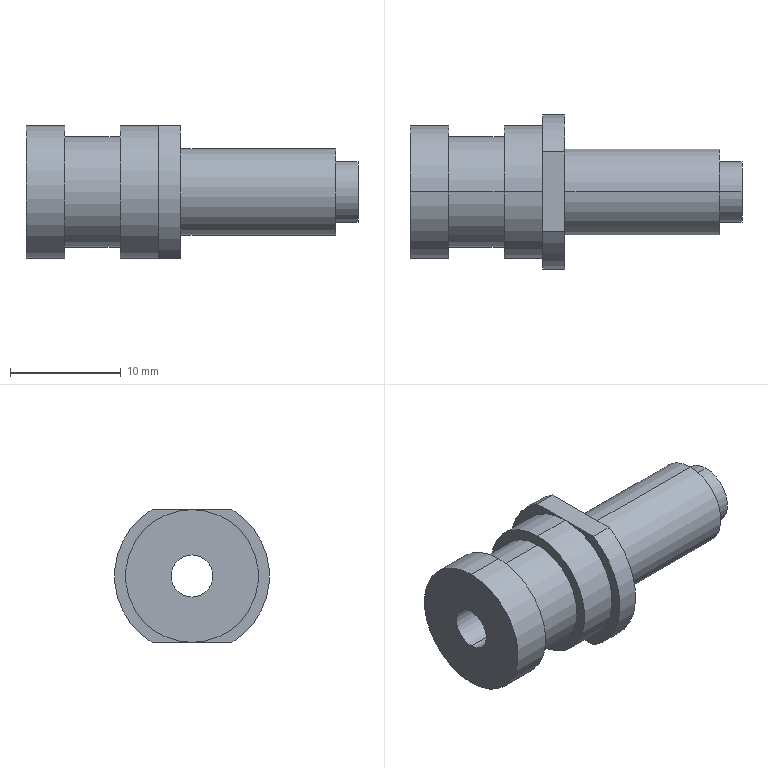Component | SolidWorks | Connector-1 | 1 solid | 24 faces | box 30 x 14 x 12 mm | volume 1849 mm3 | cylinder 14 | plane 10 | commonest cylinder face diameters 12 x4 10 x2 5.5 x2 3.8 x2 7.8 x2 14 x2
build123d program:
from build123d import *

# Parameters (mm, degrees)
SKETCH1_R           = 3.9
BOSS_EXTRUDE1_DEPTH = 16
SKETCH2_R           = 7
BOSS_EXTRUDE2_DEPTH = 14
SKETCH3_R           = 1.9
CUT_EXTRUDE1_DEPTH  = 32.591
CHAMFER1_SIZE       = 1
CUT_EXTRUDE2_START  = -12
SKETCH4_R           = 7
SKETCH4_R_2         = 6
CUT_EXTRUDE2_DEPTH  = 12
SKETCH6_R           = 4.5
SKETCH6_R_2         = 2.75
CUT_EXTRUDE4_DEPTH  = 2
SKETCH8_W           = 1
SKETCH8_H           = 5
CUT_EXTRUDE5_DEPTH  = 19.815


with BuildPart() as part:
    # Sketch1 → Boss-Extrude1 (new body)
    with BuildSketch(Plane.XY):
        Circle(SKETCH1_R)
    extrude(amount=BOSS_EXTRUDE1_DEPTH)

    # Sketch2 → Boss-Extrude2 (add)
    with BuildSketch(Plane.XY.offset(16)):
        Circle(SKETCH2_R)
    extrude(amount=BOSS_EXTRUDE2_DEPTH)

    # Sketch3 → Cut-Extrude1 (cut, through all)
    with BuildSketch(Plane(origin=(0, 0, 0), x_dir=(-1, 0, 0), z_dir=(0, 0, -1))):
        Circle(SKETCH3_R)
    extrude(amount=-CUT_EXTRUDE1_DEPTH, mode=Mode.SUBTRACT)

    # Chamfer1
    chamfer1_edges = [part.edges().sort_by_distance(p)[0] for p in [
        (-3.9, 0, 0),
    ]]
    chamfer(chamfer1_edges, length=CHAMFER1_SIZE)

    # Sketch4 → Cut-Extrude2 (cut)
    with BuildSketch(Plane.XY.offset(30).offset(CUT_EXTRUDE2_START)):
        Circle(SKETCH4_R)
        Circle(SKETCH4_R_2, mode=Mode.SUBTRACT)
    extrude(amount=CUT_EXTRUDE2_DEPTH, mode=Mode.SUBTRACT)

    # Sketch6 → Cut-Extrude4 (cut)
    with BuildSketch(Plane(origin=(0, 0, 0), x_dir=(-1, 0, 0), z_dir=(0, 0, -1))):
        Circle(SKETCH6_R)
        Circle(SKETCH6_R_2, mode=Mode.SUBTRACT)
    extrude(amount=-CUT_EXTRUDE4_DEPTH, mode=Mode.SUBTRACT)

    # Sketch8 → Cut-Revolve1 (revolve, cut)
    with BuildSketch(Plane(origin=(0, 0, 0), x_dir=(1, 0, 0), z_dir=(0, 1, 0)), mode=Mode.PRIVATE) as cut_revolve1_sk:
        with Locations((-5.5, -24)):
            Rectangle(SKETCH8_W, SKETCH8_H)
    revolve(cut_revolve1_sk.sketch.rotate(Axis((0, 0, 30), (0, 0, -1)), 180), axis=Axis((0, 0, 30), (0, 0, -1)), mode=Mode.SUBTRACT)

    # Sketch9 → Cut-Extrude5 (cut, through all)
    with BuildSketch(Plane(origin=(0, 0, 16), x_dir=(-1, 0, 0), z_dir=(0, 0, -1))):
        with BuildLine():
            Line((-6, 3.606), (-6, -3.606))
            ThreePointArc((-6, -3.606), (-7, 0), (-6, 3.606))
        make_face()
        with BuildLine():
            Line((6, 3.606), (6, -3.606))
            ThreePointArc((6, -3.606), (7, 0), (6, 3.606))
        make_face()
    extrude(amount=-CUT_EXTRUDE5_DEPTH, mode=Mode.SUBTRACT)


solid = part.part

# Placed as in the assembly
solid = solid.moved(Location((20.76, 74.679, 11), (0, -90, 0)))
STEP:
#1=CARTESIAN_POINT('',(-0.02914,2.94,0.6299));
#2=VERTEX_POINT('',#1);
#3=CARTESIAN_POINT('',(-0.02914,2.94,0.2362));
#4=VERTEX_POINT('',#3);
#5=CARTESIAN_POINT('',(-0.02914,2.94,0.4331));
#6=DIRECTION('',(-1.,-0.,-0.));
#7=DIRECTION('',(-0.,0.,1.));
#8=AXIS2_PLACEMENT_3D('',#5,#6,#7);
#9=CIRCLE('',#8,0.1969);
#10=EDGE_CURVE('',#2,#4,#9,.T.);
#11=ORIENTED_EDGE('',*,*,#10,.T.);
#12=CARTESIAN_POINT('',(-0.226,2.94,0.2362));
#13=VERTEX_POINT('',#12);
#14=CARTESIAN_POINT('',(-0.3638,2.94,0.2362));
#15=DIRECTION('',(-1.,-0.,-0.));
#16=VECTOR('',#15,39.37);
#17=LINE('',#14,#16);
#18=EDGE_CURVE('',#4,#13,#17,.T.);
#19=ORIENTED_EDGE('',*,*,#18,.T.);
#20=CARTESIAN_POINT('',(-0.226,2.94,0.6299));
#21=VERTEX_POINT('',#20);
#22=CARTESIAN_POINT('',(-0.226,2.94,0.4331));
#23=DIRECTION('',(-1.,-0.,-0.));
#24=DIRECTION('',(-0.,0.,1.));
#25=AXIS2_PLACEMENT_3D('',#22,#23,#24);
#26=CIRCLE('',#25,0.1969);
#27=EDGE_CURVE('',#21,#13,#26,.T.);
#28=ORIENTED_EDGE('',*,*,#27,.F.);
#29=CARTESIAN_POINT('',(-0.3638,2.94,0.6299));
#30=DIRECTION('',(-1.,-0.,-0.));
#31=VECTOR('',#30,39.37);
#32=LINE('',#29,#31);
#33=EDGE_CURVE('',#2,#21,#32,.T.);
#34=ORIENTED_EDGE('',*,*,#33,.F.);
#35=EDGE_LOOP('',(#11,#19,#28,#34));
#36=FACE_OUTER_BOUND('',#35,.T.);
#37=CARTESIAN_POINT('',(-0.3638,2.94,0.4331));
#38=DIRECTION('',(-1.,-0.,-0.));
#39=DIRECTION('',(-0.,0.,1.));
#40=AXIS2_PLACEMENT_3D('',#37,#38,#39);
#41=CYLINDRICAL_SURFACE('',#40,0.1969);
#42=ADVANCED_FACE('',(#36),#41,.T.);
#43=CARTESIAN_POINT('',(0.7386,2.94,0.3248));
#44=VERTEX_POINT('',#43);
#45=CARTESIAN_POINT('',(0.7386,2.94,0.5413));
#46=VERTEX_POINT('',#45);
#47=CARTESIAN_POINT('',(0.7386,2.94,0.4331));
#48=DIRECTION('',(1.,0.,0.));
#49=DIRECTION('',(0.,0.,-1.));
#50=AXIS2_PLACEMENT_3D('',#47,#48,#49);
#51=CIRCLE('',#50,0.1083);
#52=EDGE_CURVE('',#44,#46,#51,.T.);
#53=ORIENTED_EDGE('',*,*,#52,.T.);
#54=CARTESIAN_POINT('',(0.8173,2.94,0.5413));
#55=VERTEX_POINT('',#54);
#56=CARTESIAN_POINT('',(0.7386,2.94,0.5413));
#57=DIRECTION('',(1.,0.,0.));
#58=VECTOR('',#57,39.37);
#59=LINE('',#56,#58);
#60=EDGE_CURVE('',#46,#55,#59,.T.);
#61=ORIENTED_EDGE('',*,*,#60,.T.);
#62=CARTESIAN_POINT('',(0.8173,2.94,0.3248));
#63=VERTEX_POINT('',#62);
#64=CARTESIAN_POINT('',(0.8173,2.94,0.4331));
#65=DIRECTION('',(1.,0.,0.));
#66=DIRECTION('',(0.,0.,-1.));
#67=AXIS2_PLACEMENT_3D('',#64,#65,#66);
#68=CIRCLE('',#67,0.1083);
#69=EDGE_CURVE('',#63,#55,#68,.T.);
#70=ORIENTED_EDGE('',*,*,#69,.F.);
#71=CARTESIAN_POINT('',(0.7386,2.94,0.3248));
#72=DIRECTION('',(1.,0.,0.));
#73=VECTOR('',#72,39.37);
#74=LINE('',#71,#73);
#75=EDGE_CURVE('',#44,#63,#74,.T.);
#76=ORIENTED_EDGE('',*,*,#75,.F.);
#77=EDGE_LOOP('',(#53,#61,#70,#76));
#78=FACE_OUTER_BOUND('',#77,.T.);
#79=CARTESIAN_POINT('',(0.7386,2.94,0.4331));
#80=DIRECTION('',(1.,0.,0.));
#81=DIRECTION('',(0.,0.,-1.));
#82=AXIS2_PLACEMENT_3D('',#79,#80,#81);
#83=CYLINDRICAL_SURFACE('',#82,0.1083);
#84=ADVANCED_FACE('',(#78),#83,.T.);
#85=CARTESIAN_POINT('',(-0.3638,2.94,0.5079));
#86=VERTEX_POINT('',#85);
#87=CARTESIAN_POINT('',(-0.3638,2.94,0.3583));
#88=VERTEX_POINT('',#87);
#89=CARTESIAN_POINT('',(-0.3638,2.94,0.4331));
#90=DIRECTION('',(1.,0.,0.));
#91=DIRECTION('',(0.,0.,-1.));
#92=AXIS2_PLACEMENT_3D('',#89,#90,#91);
#93=CIRCLE('',#92,0.0748);
#94=EDGE_CURVE('',#86,#88,#93,.T.);
#95=ORIENTED_EDGE('',*,*,#94,.F.);
#96=CARTESIAN_POINT('',(0.8173,2.94,0.5079));
#97=VERTEX_POINT('',#96);
#98=CARTESIAN_POINT('',(-0.3638,2.94,0.5079));
#99=DIRECTION('',(1.,0.,0.));
#100=VECTOR('',#99,39.37);
#101=LINE('',#98,#100);
#102=EDGE_CURVE('',#86,#97,#101,.T.);
#103=ORIENTED_EDGE('',*,*,#102,.T.);
#104=CARTESIAN_POINT('',(0.8173,2.94,0.3583));
#105=VERTEX_POINT('',#104);
#106=CARTESIAN_POINT('',(0.8173,2.94,0.4331));
#107=DIRECTION('',(1.,0.,0.));
#108=DIRECTION('',(0.,0.,-1.));
#109=AXIS2_PLACEMENT_3D('',#106,#107,#108);
#110=CIRCLE('',#109,0.0748);
#111=EDGE_CURVE('',#97,#105,#110,.T.);
#112=ORIENTED_EDGE('',*,*,#111,.T.);
#113=CARTESIAN_POINT('',(-0.3638,2.94,0.3583));
#114=DIRECTION('',(1.,0.,0.));
#115=VECTOR('',#114,39.37);
#116=LINE('',#113,#115);
#117=EDGE_CURVE('',#88,#105,#116,.T.);
#118=ORIENTED_EDGE('',*,*,#117,.F.);
#119=EDGE_LOOP('',(#95,#103,#112,#118));
#120=FACE_OUTER_BOUND('',#119,.T.);
#121=CARTESIAN_POINT('',(-0.3638,2.94,0.4331));
#122=DIRECTION('',(1.,0.,0.));
#123=DIRECTION('',(0.,0.,-1.));
#124=AXIS2_PLACEMENT_3D('',#121,#122,#123);
#125=CYLINDRICAL_SURFACE('',#124,0.0748);
#126=ADVANCED_FACE('',(#120),#125,.F.);
#127=CARTESIAN_POINT('',(0.1874,2.94,0.5866));
#128=VERTEX_POINT('',#127);
#129=CARTESIAN_POINT('',(0.1874,2.94,0.2795));
#130=VERTEX_POINT('',#129);
#131=CARTESIAN_POINT('',(0.1874,2.94,0.4331));
#132=DIRECTION('',(-1.,-0.,-0.));
#133=DIRECTION('',(-0.,0.,1.));
#134=AXIS2_PLACEMENT_3D('',#131,#132,#133);
#135=CIRCLE('',#134,0.1535);
#136=EDGE_CURVE('',#128,#130,#135,.T.);
#137=ORIENTED_EDGE('',*,*,#136,.F.);
#138=CARTESIAN_POINT('',(0.7386,2.94,0.5866));
#139=VERTEX_POINT('',#138);
#140=CARTESIAN_POINT('',(0.1874,2.94,0.5866));
#141=DIRECTION('',(1.,0.,0.));
#142=VECTOR('',#141,39.37);
#143=LINE('',#140,#142);
#144=EDGE_CURVE('',#128,#139,#143,.T.);
#145=ORIENTED_EDGE('',*,*,#144,.T.);
#146=CARTESIAN_POINT('',(0.7386,2.94,0.2795));
#147=VERTEX_POINT('',#146);
#148=CARTESIAN_POINT('',(0.7386,2.94,0.4331));
#149=DIRECTION('',(1.,0.,0.));
#150=DIRECTION('',(0.,0.,-1.));
#151=AXIS2_PLACEMENT_3D('',#148,#149,#150);
#152=CIRCLE('',#151,0.1535);
#153=EDGE_CURVE('',#147,#139,#152,.T.);
#154=ORIENTED_EDGE('',*,*,#153,.F.);
#155=CARTESIAN_POINT('',(0.1874,2.94,0.2795));
#156=DIRECTION('',(1.,0.,0.));
#157=VECTOR('',#156,39.37);
#158=LINE('',#155,#157);
#159=EDGE_CURVE('',#130,#147,#158,.T.);
#160=ORIENTED_EDGE('',*,*,#159,.F.);
#161=EDGE_LOOP('',(#137,#145,#154,#160));
#162=FACE_OUTER_BOUND('',#161,.T.);
#163=CARTESIAN_POINT('',(0.1874,2.94,0.4331));
#164=DIRECTION('',(1.,0.,0.));
#165=DIRECTION('',(0.,0.,-1.));
#166=AXIS2_PLACEMENT_3D('',#163,#164,#165);
#167=CYLINDRICAL_SURFACE('',#166,0.1535);
#168=ADVANCED_FACE('',(#162),#167,.T.);
#169=CARTESIAN_POINT('',(0.1087,2.94,0.6693));
#170=VERTEX_POINT('',#169);
#171=CARTESIAN_POINT('',(0.1087,2.94,0.1969));
#172=VERTEX_POINT('',#171);
#173=CARTESIAN_POINT('',(0.1087,2.94,0.4331));
#174=DIRECTION('',(-1.,-0.,-0.));
#175=DIRECTION('',(-0.,0.,1.));
#176=AXIS2_PLACEMENT_3D('',#173,#174,#175);
#177=CIRCLE('',#176,0.2362);
#178=EDGE_CURVE('',#170,#172,#177,.T.);
#179=ORIENTED_EDGE('',*,*,#178,.T.);
#180=CARTESIAN_POINT('',(-0.02914,2.94,0.1969));
#181=VERTEX_POINT('',#180);
#182=CARTESIAN_POINT('',(0.1087,2.94,0.1969));
#183=DIRECTION('',(-1.,-0.,-0.));
#184=VECTOR('',#183,39.37);
#185=LINE('',#182,#184);
#186=EDGE_CURVE('',#172,#181,#185,.T.);
#187=ORIENTED_EDGE('',*,*,#186,.T.);
#188=CARTESIAN_POINT('',(-0.02914,2.94,0.6693));
#189=VERTEX_POINT('',#188);
#190=CARTESIAN_POINT('',(-0.02914,2.94,0.4331));
#191=DIRECTION('',(-1.,-0.,-0.));
#192=DIRECTION('',(-0.,0.,1.));
#193=AXIS2_PLACEMENT_3D('',#190,#191,#192);
#194=CIRCLE('',#193,0.2362);
#195=EDGE_CURVE('',#189,#181,#194,.T.);
#196=ORIENTED_EDGE('',*,*,#195,.F.);
#197=CARTESIAN_POINT('',(0.1087,2.94,0.6693));
#198=DIRECTION('',(-1.,-0.,-0.));
#199=VECTOR('',#198,39.37);
#200=LINE('',#197,#199);
#201=EDGE_CURVE('',#170,#189,#200,.T.);
#202=ORIENTED_EDGE('',*,*,#201,.F.);
#203=EDGE_LOOP('',(#179,#187,#196,#202));
#204=FACE_OUTER_BOUND('',#203,.T.);
#205=CARTESIAN_POINT('',(0.1087,2.94,0.4331));
#206=DIRECTION('',(-1.,-0.,-0.));
#207=DIRECTION('',(-0.,0.,1.));
#208=AXIS2_PLACEMENT_3D('',#205,#206,#207);
#209=CYLINDRICAL_SURFACE('',#208,0.2362);
#210=ADVANCED_FACE('',(#204),#209,.T.);
#211=CARTESIAN_POINT('',(-0.226,2.94,0.6693));
#212=VERTEX_POINT('',#211);
#213=CARTESIAN_POINT('',(-0.226,2.94,0.1969));
#214=VERTEX_POINT('',#213);
#215=CARTESIAN_POINT('',(-0.226,2.94,0.4331));
#216=DIRECTION('',(-1.,-0.,-0.));
#217=DIRECTION('',(-0.,0.,1.));
#218=AXIS2_PLACEMENT_3D('',#215,#216,#217);
#219=CIRCLE('',#218,0.2362);
#220=EDGE_CURVE('',#212,#214,#219,.T.);
#221=ORIENTED_EDGE('',*,*,#220,.T.);
#222=CARTESIAN_POINT('',(-0.3638,2.94,0.1969));
#223=VERTEX_POINT('',#222);
#224=CARTESIAN_POINT('',(0.1087,2.94,0.1969));
#225=DIRECTION('',(-1.,-0.,-0.));
#226=VECTOR('',#225,39.37);
#227=LINE('',#224,#226);
#228=EDGE_CURVE('',#214,#223,#227,.T.);
#229=ORIENTED_EDGE('',*,*,#228,.T.);
#230=CARTESIAN_POINT('',(-0.3638,2.94,0.6693));
#231=VERTEX_POINT('',#230);
#232=CARTESIAN_POINT('',(-0.3638,2.94,0.4331));
#233=DIRECTION('',(-1.,-0.,-0.));
#234=DIRECTION('',(-0.,0.,1.));
#235=AXIS2_PLACEMENT_3D('',#232,#233,#234);
#236=CIRCLE('',#235,0.2362);
#237=EDGE_CURVE('',#231,#223,#236,.T.);
#238=ORIENTED_EDGE('',*,*,#237,.F.);
#239=CARTESIAN_POINT('',(0.1087,2.94,0.6693));
#240=DIRECTION('',(-1.,-0.,-0.));
#241=VECTOR('',#240,39.37);
#242=LINE('',#239,#241);
#243=EDGE_CURVE('',#212,#231,#242,.T.);
#244=ORIENTED_EDGE('',*,*,#243,.F.);
#245=EDGE_LOOP('',(#221,#229,#238,#244));
#246=FACE_OUTER_BOUND('',#245,.T.);
#247=CARTESIAN_POINT('',(0.1087,2.94,0.4331));
#248=DIRECTION('',(-1.,-0.,-0.));
#249=DIRECTION('',(-0.,0.,1.));
#250=AXIS2_PLACEMENT_3D('',#247,#248,#249);
#251=CYLINDRICAL_SURFACE('',#250,0.2362);
#252=ADVANCED_FACE('',(#246),#251,.T.);
#253=CARTESIAN_POINT('',(0.1087,2.798,0.1969));
#254=VERTEX_POINT('',#253);
#255=CARTESIAN_POINT('',(0.1087,2.798,0.6693));
#256=VERTEX_POINT('',#255);
#257=CARTESIAN_POINT('',(0.1087,2.94,0.4331));
#258=DIRECTION('',(-1.,-0.,-0.));
#259=DIRECTION('',(-0.,0.,1.));
#260=AXIS2_PLACEMENT_3D('',#257,#258,#259);
#261=CIRCLE('',#260,0.2756);
#262=EDGE_CURVE('',#254,#256,#261,.T.);
#263=ORIENTED_EDGE('',*,*,#262,.F.);
#264=CARTESIAN_POINT('',(0.1874,2.798,0.1969));
#265=VERTEX_POINT('',#264);
#266=CARTESIAN_POINT('',(-0.3638,2.798,0.1969));
#267=DIRECTION('',(1.,0.,0.));
#268=VECTOR('',#267,39.37);
#269=LINE('',#266,#268);
#270=EDGE_CURVE('',#254,#265,#269,.T.);
#271=ORIENTED_EDGE('',*,*,#270,.T.);
#272=CARTESIAN_POINT('',(0.1874,2.798,0.6693));
#273=VERTEX_POINT('',#272);
#274=CARTESIAN_POINT('',(0.1874,2.94,0.4331));
#275=DIRECTION('',(-1.,-0.,-0.));
#276=DIRECTION('',(-0.,0.,1.));
#277=AXIS2_PLACEMENT_3D('',#274,#275,#276);
#278=CIRCLE('',#277,0.2756);
#279=EDGE_CURVE('',#265,#273,#278,.T.);
#280=ORIENTED_EDGE('',*,*,#279,.T.);
#281=CARTESIAN_POINT('',(-0.3638,2.798,0.6693));
#282=DIRECTION('',(1.,0.,0.));
#283=VECTOR('',#282,39.37);
#284=LINE('',#281,#283);
#285=EDGE_CURVE('',#256,#273,#284,.T.);
#286=ORIENTED_EDGE('',*,*,#285,.F.);
#287=EDGE_LOOP('',(#263,#271,#280,#286));
#288=FACE_OUTER_BOUND('',#287,.T.);
#289=CARTESIAN_POINT('',(-0.3638,2.94,0.4331));
#290=DIRECTION('',(1.,0.,0.));
#291=DIRECTION('',(0.,0.,-1.));
#292=AXIS2_PLACEMENT_3D('',#289,#290,#291);
#293=CYLINDRICAL_SURFACE('',#292,0.2756);
#294=ADVANCED_FACE('',(#288),#293,.T.);
#295=CARTESIAN_POINT('',(0.1087,2.94,0.1969));
#296=DIRECTION('',(-0.,1.,0.));
#297=VECTOR('',#296,39.37);
#298=LINE('',#295,#297);
#299=EDGE_CURVE('',#254,#172,#298,.T.);
#300=ORIENTED_EDGE('',*,*,#299,.F.);
#301=ORIENTED_EDGE('',*,*,#262,.T.);
#302=CARTESIAN_POINT('',(0.1087,2.94,0.6693));
#303=DIRECTION('',(0.,-1.,0.));
#304=VECTOR('',#303,39.37);
#305=LINE('',#302,#304);
#306=EDGE_CURVE('',#170,#256,#305,.T.);
#307=ORIENTED_EDGE('',*,*,#306,.F.);
#308=CARTESIAN_POINT('',(0.1087,2.94,0.4331));
#309=DIRECTION('',(-1.,-0.,-0.));
#310=DIRECTION('',(-0.,0.,1.));
#311=AXIS2_PLACEMENT_3D('',#308,#309,#310);
#312=CIRCLE('',#311,0.2362);
#313=EDGE_CURVE('',#172,#170,#312,.T.);
#314=ORIENTED_EDGE('',*,*,#313,.F.);
#315=EDGE_LOOP('',(#300,#301,#307,#314));
#316=FACE_OUTER_BOUND('',#315,.T.);
#317=CARTESIAN_POINT('',(0.1087,2.94,0.4331));
#318=DIRECTION('',(-1.,-0.,-0.));
#319=DIRECTION('',(-0.,0.,1.));
#320=AXIS2_PLACEMENT_3D('',#317,#318,#319);
#321=PLANE('',#320);
#322=ADVANCED_FACE('',(#316),#321,.T.);
#323=ORIENTED_EDGE('',*,*,#228,.F.);
#324=CARTESIAN_POINT('',(-0.226,2.94,0.4331));
#325=DIRECTION('',(-1.,-0.,-0.));
#326=DIRECTION('',(-0.,0.,1.));
#327=AXIS2_PLACEMENT_3D('',#324,#325,#326);
#328=CIRCLE('',#327,0.2362);
#329=EDGE_CURVE('',#214,#212,#328,.T.);
#330=ORIENTED_EDGE('',*,*,#329,.T.);
#331=ORIENTED_EDGE('',*,*,#243,.T.);
#332=CARTESIAN_POINT('',(-0.3638,2.94,0.4331));
#333=DIRECTION('',(-1.,-0.,-0.));
#334=DIRECTION('',(-0.,0.,1.));
#335=AXIS2_PLACEMENT_3D('',#332,#333,#334);
#336=CIRCLE('',#335,0.2362);
#337=EDGE_CURVE('',#223,#231,#336,.T.);
#338=ORIENTED_EDGE('',*,*,#337,.F.);
#339=EDGE_LOOP('',(#323,#330,#331,#338));
#340=FACE_OUTER_BOUND('',#339,.T.);
#341=CARTESIAN_POINT('',(0.1087,2.94,0.4331));
#342=DIRECTION('',(-1.,-0.,-0.));
#343=DIRECTION('',(-0.,0.,1.));
#344=AXIS2_PLACEMENT_3D('',#341,#342,#343);
#345=CYLINDRICAL_SURFACE('',#344,0.2362);
#346=ADVANCED_FACE('',(#340),#345,.T.);
#347=ORIENTED_EDGE('',*,*,#186,.F.);
#348=ORIENTED_EDGE('',*,*,#313,.T.);
#349=ORIENTED_EDGE('',*,*,#201,.T.);
#350=CARTESIAN_POINT('',(-0.02914,2.94,0.4331));
#351=DIRECTION('',(-1.,-0.,-0.));
#352=DIRECTION('',(-0.,0.,1.));
#353=AXIS2_PLACEMENT_3D('',#350,#351,#352);
#354=CIRCLE('',#353,0.2362);
#355=EDGE_CURVE('',#181,#189,#354,.T.);
#356=ORIENTED_EDGE('',*,*,#355,.F.);
#357=EDGE_LOOP('',(#347,#348,#349,#356));
#358=FACE_OUTER_BOUND('',#357,.T.);
#359=CARTESIAN_POINT('',(0.1087,2.94,0.4331));
#360=DIRECTION('',(-1.,-0.,-0.));
#361=DIRECTION('',(-0.,0.,1.));
#362=AXIS2_PLACEMENT_3D('',#359,#360,#361);
#363=CYLINDRICAL_SURFACE('',#362,0.2362);
#364=ADVANCED_FACE('',(#358),#363,.T.);
#365=ORIENTED_EDGE('',*,*,#144,.F.);
#366=CARTESIAN_POINT('',(0.1874,2.94,0.4331));
#367=DIRECTION('',(-1.,-0.,-0.));
#368=DIRECTION('',(-0.,0.,1.));
#369=AXIS2_PLACEMENT_3D('',#366,#367,#368);
#370=CIRCLE('',#369,0.1535);
#371=EDGE_CURVE('',#130,#128,#370,.T.);
#372=ORIENTED_EDGE('',*,*,#371,.F.);
#373=ORIENTED_EDGE('',*,*,#159,.T.);
#374=CARTESIAN_POINT('',(0.7386,2.94,0.4331));
#375=DIRECTION('',(1.,0.,0.));
#376=DIRECTION('',(0.,0.,-1.));
#377=AXIS2_PLACEMENT_3D('',#374,#375,#376);
#378=CIRCLE('',#377,0.1535);
#379=EDGE_CURVE('',#139,#147,#378,.T.);
#380=ORIENTED_EDGE('',*,*,#379,.F.);
#381=EDGE_LOOP('',(#365,#372,#373,#380));
#382=FACE_OUTER_BOUND('',#381,.T.);
#383=CARTESIAN_POINT('',(0.1874,2.94,0.4331));
#384=DIRECTION('',(1.,0.,0.));
#385=DIRECTION('',(0.,0.,-1.));
#386=AXIS2_PLACEMENT_3D('',#383,#384,#385);
#387=CYLINDRICAL_SURFACE('',#386,0.1535);
#388=ADVANCED_FACE('',(#382),#387,.T.);
#389=CARTESIAN_POINT('',(0.8173,2.94,0.4331));
#390=DIRECTION('',(1.,0.,0.));
#391=DIRECTION('',(0.,0.,-1.));
#392=AXIS2_PLACEMENT_3D('',#389,#390,#391);
#393=CIRCLE('',#392,0.0748);
#394=EDGE_CURVE('',#105,#97,#393,.T.);
#395=ORIENTED_EDGE('',*,*,#394,.F.);
#396=ORIENTED_EDGE('',*,*,#111,.F.);
#397=EDGE_LOOP('',(#395,#396));
#398=FACE_BOUND('',#397,.T.);
#399=ORIENTED_EDGE('',*,*,#69,.T.);
#400=CARTESIAN_POINT('',(0.8173,2.94,0.4331));
#401=DIRECTION('',(1.,0.,0.));
#402=DIRECTION('',(0.,0.,-1.));
#403=AXIS2_PLACEMENT_3D('',#400,#401,#402);
#404=CIRCLE('',#403,0.1083);
#405=EDGE_CURVE('',#55,#63,#404,.T.);
#406=ORIENTED_EDGE('',*,*,#405,.T.);
#407=EDGE_LOOP('',(#399,#406));
#408=FACE_OUTER_BOUND('',#407,.T.);
#409=CARTESIAN_POINT('',(0.8173,2.94,0.4331));
#410=DIRECTION('',(-1.,-0.,-0.));
#411=DIRECTION('',(-0.,0.,1.));
#412=AXIS2_PLACEMENT_3D('',#409,#410,#411);
#413=PLANE('',#412);
#414=ADVANCED_FACE('',(#398,#408),#413,.F.);
#415=CARTESIAN_POINT('',(0.1874,3.082,0.6693));
#416=VERTEX_POINT('',#415);
#417=CARTESIAN_POINT('',(0.1874,3.082,0.1969));
#418=VERTEX_POINT('',#417);
#419=CARTESIAN_POINT('',(0.1874,2.94,0.4331));
#420=DIRECTION('',(-1.,-0.,-0.));
#421=DIRECTION('',(-0.,0.,1.));
#422=AXIS2_PLACEMENT_3D('',#419,#420,#421);
#423=CIRCLE('',#422,0.2756);
#424=EDGE_CURVE('',#416,#418,#423,.T.);
#425=ORIENTED_EDGE('',*,*,#424,.T.);
#426=CARTESIAN_POINT('',(0.1087,3.082,0.1969));
#427=VERTEX_POINT('',#426);
#428=CARTESIAN_POINT('',(-0.3638,3.082,0.1969));
#429=DIRECTION('',(1.,0.,0.));
#430=VECTOR('',#429,39.37);
#431=LINE('',#428,#430);
#432=EDGE_CURVE('',#427,#418,#431,.T.);
#433=ORIENTED_EDGE('',*,*,#432,.F.);
#434=CARTESIAN_POINT('',(0.1087,3.082,0.6693));
#435=VERTEX_POINT('',#434);
#436=CARTESIAN_POINT('',(0.1087,2.94,0.4331));
#437=DIRECTION('',(-1.,-0.,-0.));
#438=DIRECTION('',(-0.,0.,1.));
#439=AXIS2_PLACEMENT_3D('',#436,#437,#438);
#440=CIRCLE('',#439,0.2756);
#441=EDGE_CURVE('',#435,#427,#440,.T.);
#442=ORIENTED_EDGE('',*,*,#441,.F.);
#443=CARTESIAN_POINT('',(-0.3638,3.082,0.6693));
#444=DIRECTION('',(1.,0.,0.));
#445=VECTOR('',#444,39.37);
#446=LINE('',#443,#445);
#447=EDGE_CURVE('',#435,#416,#446,.T.);
#448=ORIENTED_EDGE('',*,*,#447,.T.);
#449=EDGE_LOOP('',(#425,#433,#442,#448));
#450=FACE_OUTER_BOUND('',#449,.T.);
#451=CARTESIAN_POINT('',(-0.3638,2.94,0.4331));
#452=DIRECTION('',(1.,0.,0.));
#453=DIRECTION('',(0.,0.,-1.));
#454=AXIS2_PLACEMENT_3D('',#451,#452,#453);
#455=CYLINDRICAL_SURFACE('',#454,0.2756);
#456=ADVANCED_FACE('',(#450),#455,.T.);
#457=CARTESIAN_POINT('',(-0.3638,2.94,0.4331));
#458=DIRECTION('',(1.,0.,0.));
#459=DIRECTION('',(0.,0.,-1.));
#460=AXIS2_PLACEMENT_3D('',#457,#458,#459);
#461=CIRCLE('',#460,0.0748);
#462=EDGE_CURVE('',#88,#86,#461,.T.);
#463=ORIENTED_EDGE('',*,*,#462,.T.);
#464=ORIENTED_EDGE('',*,*,#94,.T.);
#465=EDGE_LOOP('',(#463,#464));
#466=FACE_BOUND('',#465,.T.);
#467=ORIENTED_EDGE('',*,*,#237,.T.);
#468=ORIENTED_EDGE('',*,*,#337,.T.);
#469=EDGE_LOOP('',(#467,#468));
#470=FACE_OUTER_BOUND('',#469,.T.);
#471=CARTESIAN_POINT('',(-0.3638,2.94,0.4331));
#472=DIRECTION('',(-1.,-0.,-0.));
#473=DIRECTION('',(-0.,0.,1.));
#474=AXIS2_PLACEMENT_3D('',#471,#472,#473);
#475=PLANE('',#474);
#476=ADVANCED_FACE('',(#466,#470),#475,.T.);
#477=ORIENTED_EDGE('',*,*,#279,.F.);
#478=CARTESIAN_POINT('',(0.1874,3.082,0.1969));
#479=DIRECTION('',(0.,-1.,0.));
#480=VECTOR('',#479,39.37);
#481=LINE('',#478,#480);
#482=EDGE_CURVE('',#418,#265,#481,.T.);
#483=ORIENTED_EDGE('',*,*,#482,.F.);
#484=ORIENTED_EDGE('',*,*,#424,.F.);
#485=CARTESIAN_POINT('',(0.1874,3.082,0.6693));
#486=DIRECTION('',(-0.,1.,0.));
#487=VECTOR('',#486,39.37);
#488=LINE('',#485,#487);
#489=EDGE_CURVE('',#273,#416,#488,.T.);
#490=ORIENTED_EDGE('',*,*,#489,.F.);
#491=EDGE_LOOP('',(#477,#483,#484,#490));
#492=FACE_OUTER_BOUND('',#491,.T.);
#493=ORIENTED_EDGE('',*,*,#371,.T.);
#494=ORIENTED_EDGE('',*,*,#136,.T.);
#495=EDGE_LOOP('',(#493,#494));
#496=FACE_BOUND('',#495,.T.);
#497=CARTESIAN_POINT('',(0.1874,2.94,0.4331));
#498=DIRECTION('',(-1.,-0.,-0.));
#499=DIRECTION('',(-0.,0.,1.));
#500=AXIS2_PLACEMENT_3D('',#497,#498,#499);
#501=PLANE('',#500);
#502=ADVANCED_FACE('',(#492,#496),#501,.F.);
#503=ORIENTED_EDGE('',*,*,#102,.F.);
#504=ORIENTED_EDGE('',*,*,#462,.F.);
#505=ORIENTED_EDGE('',*,*,#117,.T.);
#506=ORIENTED_EDGE('',*,*,#394,.T.);
#507=EDGE_LOOP('',(#503,#504,#505,#506));
#508=FACE_OUTER_BOUND('',#507,.T.);
#509=CARTESIAN_POINT('',(-0.3638,2.94,0.4331));
#510=DIRECTION('',(1.,0.,0.));
#511=DIRECTION('',(0.,0.,-1.));
#512=AXIS2_PLACEMENT_3D('',#509,#510,#511);
#513=CYLINDRICAL_SURFACE('',#512,0.0748);
#514=ADVANCED_FACE('',(#508),#513,.F.);
#515=CARTESIAN_POINT('',(0.1087,2.94,0.1969));
#516=DIRECTION('',(-0.,1.,0.));
#517=VECTOR('',#516,39.37);
#518=LINE('',#515,#517);
#519=EDGE_CURVE('',#172,#427,#518,.T.);
#520=ORIENTED_EDGE('',*,*,#519,.F.);
#521=ORIENTED_EDGE('',*,*,#178,.F.);
#522=CARTESIAN_POINT('',(0.1087,2.94,0.6693));
#523=DIRECTION('',(0.,-1.,0.));
#524=VECTOR('',#523,39.37);
#525=LINE('',#522,#524);
#526=EDGE_CURVE('',#435,#170,#525,.T.);
#527=ORIENTED_EDGE('',*,*,#526,.F.);
#528=ORIENTED_EDGE('',*,*,#441,.T.);
#529=EDGE_LOOP('',(#520,#521,#527,#528));
#530=FACE_OUTER_BOUND('',#529,.T.);
#531=CARTESIAN_POINT('',(0.1087,2.94,0.4331));
#532=DIRECTION('',(-1.,-0.,-0.));
#533=DIRECTION('',(-0.,0.,1.));
#534=AXIS2_PLACEMENT_3D('',#531,#532,#533);
#535=PLANE('',#534);
#536=ADVANCED_FACE('',(#530),#535,.T.);
#537=ORIENTED_EDGE('',*,*,#52,.F.);
#538=CARTESIAN_POINT('',(0.7386,2.94,0.4331));
#539=DIRECTION('',(1.,0.,0.));
#540=DIRECTION('',(0.,0.,-1.));
#541=AXIS2_PLACEMENT_3D('',#538,#539,#540);
#542=CIRCLE('',#541,0.1083);
#543=EDGE_CURVE('',#46,#44,#542,.T.);
#544=ORIENTED_EDGE('',*,*,#543,.F.);
#545=EDGE_LOOP('',(#537,#544));
#546=FACE_BOUND('',#545,.T.);
#547=ORIENTED_EDGE('',*,*,#153,.T.);
#548=ORIENTED_EDGE('',*,*,#379,.T.);
#549=EDGE_LOOP('',(#547,#548));
#550=FACE_OUTER_BOUND('',#549,.T.);
#551=CARTESIAN_POINT('',(0.7386,2.94,0.4331));
#552=DIRECTION('',(1.,0.,0.));
#553=DIRECTION('',(0.,0.,-1.));
#554=AXIS2_PLACEMENT_3D('',#551,#552,#553);
#555=PLANE('',#554);
#556=ADVANCED_FACE('',(#546,#550),#555,.T.);
#557=ORIENTED_EDGE('',*,*,#60,.F.);
#558=ORIENTED_EDGE('',*,*,#543,.T.);
#559=ORIENTED_EDGE('',*,*,#75,.T.);
#560=ORIENTED_EDGE('',*,*,#405,.F.);
#561=EDGE_LOOP('',(#557,#558,#559,#560));
#562=FACE_OUTER_BOUND('',#561,.T.);
#563=CARTESIAN_POINT('',(0.7386,2.94,0.4331));
#564=DIRECTION('',(1.,0.,0.));
#565=DIRECTION('',(0.,0.,-1.));
#566=AXIS2_PLACEMENT_3D('',#563,#564,#565);
#567=CYLINDRICAL_SURFACE('',#566,0.1083);
#568=ADVANCED_FACE('',(#562),#567,.T.);
#569=ORIENTED_EDGE('',*,*,#27,.T.);
#570=CARTESIAN_POINT('',(-0.226,2.94,0.4331));
#571=DIRECTION('',(-1.,-0.,-0.));
#572=DIRECTION('',(-0.,0.,1.));
#573=AXIS2_PLACEMENT_3D('',#570,#571,#572);
#574=CIRCLE('',#573,0.1969);
#575=EDGE_CURVE('',#13,#21,#574,.T.);
#576=ORIENTED_EDGE('',*,*,#575,.T.);
#577=EDGE_LOOP('',(#569,#576));
#578=FACE_BOUND('',#577,.T.);
#579=ORIENTED_EDGE('',*,*,#220,.F.);
#580=ORIENTED_EDGE('',*,*,#329,.F.);
#581=EDGE_LOOP('',(#579,#580));
#582=FACE_OUTER_BOUND('',#581,.T.);
#583=CARTESIAN_POINT('',(-0.226,2.94,0.1969));
#584=DIRECTION('',(1.,0.,0.));
#585=DIRECTION('',(0.,0.,-1.));
#586=AXIS2_PLACEMENT_3D('',#583,#584,#585);
#587=PLANE('',#586);
#588=ADVANCED_FACE('',(#578,#582),#587,.T.);
#589=ORIENTED_EDGE('',*,*,#18,.F.);
#590=CARTESIAN_POINT('',(-0.02914,2.94,0.4331));
#591=DIRECTION('',(-1.,-0.,-0.));
#592=DIRECTION('',(-0.,0.,1.));
#593=AXIS2_PLACEMENT_3D('',#590,#591,#592);
#594=CIRCLE('',#593,0.1969);
#595=EDGE_CURVE('',#4,#2,#594,.T.);
#596=ORIENTED_EDGE('',*,*,#595,.T.);
#597=ORIENTED_EDGE('',*,*,#33,.T.);
#598=ORIENTED_EDGE('',*,*,#575,.F.);
#599=EDGE_LOOP('',(#589,#596,#597,#598));
#600=FACE_OUTER_BOUND('',#599,.T.);
#601=CARTESIAN_POINT('',(-0.3638,2.94,0.4331));
#602=DIRECTION('',(-1.,-0.,-0.));
#603=DIRECTION('',(-0.,0.,1.));
#604=AXIS2_PLACEMENT_3D('',#601,#602,#603);
#605=CYLINDRICAL_SURFACE('',#604,0.1969);
#606=ADVANCED_FACE('',(#600),#605,.T.);
#607=ORIENTED_EDGE('',*,*,#195,.T.);
#608=ORIENTED_EDGE('',*,*,#355,.T.);
#609=EDGE_LOOP('',(#607,#608));
#610=FACE_OUTER_BOUND('',#609,.T.);
#611=ORIENTED_EDGE('',*,*,#10,.F.);
#612=ORIENTED_EDGE('',*,*,#595,.F.);
#613=EDGE_LOOP('',(#611,#612));
#614=FACE_BOUND('',#613,.T.);
#615=CARTESIAN_POINT('',(-0.02914,2.94,0.1969));
#616=DIRECTION('',(-1.,-0.,-0.));
#617=DIRECTION('',(-0.,0.,1.));
#618=AXIS2_PLACEMENT_3D('',#615,#616,#617);
#619=PLANE('',#618);
#620=ADVANCED_FACE('',(#610,#614),#619,.T.);
#621=ORIENTED_EDGE('',*,*,#526,.T.);
#622=ORIENTED_EDGE('',*,*,#306,.T.);
#623=ORIENTED_EDGE('',*,*,#285,.T.);
#624=ORIENTED_EDGE('',*,*,#489,.T.);
#625=ORIENTED_EDGE('',*,*,#447,.F.);
#626=EDGE_LOOP('',(#621,#622,#623,#624,#625));
#627=FACE_OUTER_BOUND('',#626,.T.);
#628=CARTESIAN_POINT('',(-0.3638,3.082,0.6693));
#629=DIRECTION('',(0.,0.,-1.));
#630=DIRECTION('',(-1.,-0.,-0.));
#631=AXIS2_PLACEMENT_3D('',#628,#629,#630);
#632=PLANE('',#631);
#633=ADVANCED_FACE('',(#627),#632,.F.);
#634=ORIENTED_EDGE('',*,*,#299,.T.);
#635=ORIENTED_EDGE('',*,*,#519,.T.);
#636=ORIENTED_EDGE('',*,*,#432,.T.);
#637=ORIENTED_EDGE('',*,*,#482,.T.);
#638=ORIENTED_EDGE('',*,*,#270,.F.);
#639=EDGE_LOOP('',(#634,#635,#636,#637,#638));
#640=FACE_OUTER_BOUND('',#639,.T.);
#641=CARTESIAN_POINT('',(-0.3638,3.082,0.1969));
#642=DIRECTION('',(-0.,-0.,1.));
#643=DIRECTION('',(1.,0.,0.));
#644=AXIS2_PLACEMENT_3D('',#641,#642,#643);
#645=PLANE('',#644);
#646=ADVANCED_FACE('',(#640),#645,.F.);
#647=CLOSED_SHELL('',(#42,#84,#126,#168,#210,#252,#294,#322,#346,#364,#388,#414,#456,#476,#502,#514,#536,#556,#568,#588,#606,#620,#633,#646));
#648=MANIFOLD_SOLID_BREP('',#647);
#649=CARTESIAN_POINT('',(0.,0.,0.));
#650=DIRECTION('',(0.,0.,1.));
#651=DIRECTION('',(1.,0.,0.));
#652=AXIS2_PLACEMENT_3D('',#649,#650,#651);
#653=(LENGTH_UNIT()NAMED_UNIT(*)SI_UNIT($,.METRE.));
#654=LENGTH_MEASURE_WITH_UNIT(LENGTH_MEASURE(0.0254),#653);
#655=DIMENSIONAL_EXPONENTS(1.,0.,0.,0.,0.,0.,0.);
#656=(CONVERSION_BASED_UNIT('',#654)LENGTH_UNIT()NAMED_UNIT(#655));
#657=UNCERTAINTY_MEASURE_WITH_UNIT(LENGTH_MEASURE(0.00001),#656,'','');
#658=(NAMED_UNIT(*)PLANE_ANGLE_UNIT()SI_UNIT($,.RADIAN.));
#659=(NAMED_UNIT(*)SI_UNIT($,.STERADIAN.)SOLID_ANGLE_UNIT());
#660=(GEOMETRIC_REPRESENTATION_CONTEXT(3)GLOBAL_UNCERTAINTY_ASSIGNED_CONTEXT((#657))GLOBAL_UNIT_ASSIGNED_CONTEXT((#656,#658,#659))REPRESENTATION_CONTEXT('',''));
#661=ADVANCED_BREP_SHAPE_REPRESENTATION('',(#648,#652),#660);
#662=COLOUR_RGB('',0.7922,0.8196,0.9333);
#663=FILL_AREA_STYLE_COLOUR('',#662);
#664=FILL_AREA_STYLE('',(#663));
#665=SURFACE_STYLE_FILL_AREA(#664);
#666=SURFACE_SIDE_STYLE('',(#665));
#667=SURFACE_STYLE_USAGE(.BOTH.,#666);
#668=PRESENTATION_STYLE_ASSIGNMENT((#667));
#669=STYLED_ITEM('',(#668),#648);
#670=PRESENTATION_LAYER_ASSIGNMENT('','',(#669));
#671=(LENGTH_UNIT()NAMED_UNIT(*)SI_UNIT($,.METRE.));
#672=LENGTH_MEASURE_WITH_UNIT(LENGTH_MEASURE(0.0254),#671);
#673=DIMENSIONAL_EXPONENTS(1.,0.,0.,0.,0.,0.,0.);
#674=(CONVERSION_BASED_UNIT('',#672)LENGTH_UNIT()NAMED_UNIT(#673));
#675=UNCERTAINTY_MEASURE_WITH_UNIT(LENGTH_MEASURE(0.00001),#674,'','');
#676=(NAMED_UNIT(*)PLANE_ANGLE_UNIT()SI_UNIT($,.RADIAN.));
#677=(NAMED_UNIT(*)SI_UNIT($,.STERADIAN.)SOLID_ANGLE_UNIT());
#678=(GEOMETRIC_REPRESENTATION_CONTEXT(3)GLOBAL_UNCERTAINTY_ASSIGNED_CONTEXT((#675))GLOBAL_UNIT_ASSIGNED_CONTEXT((#674,#676,#677))REPRESENTATION_CONTEXT('',''));
#679=MECHANICAL_DESIGN_GEOMETRIC_PRESENTATION_REPRESENTATION('',(#669),#678);